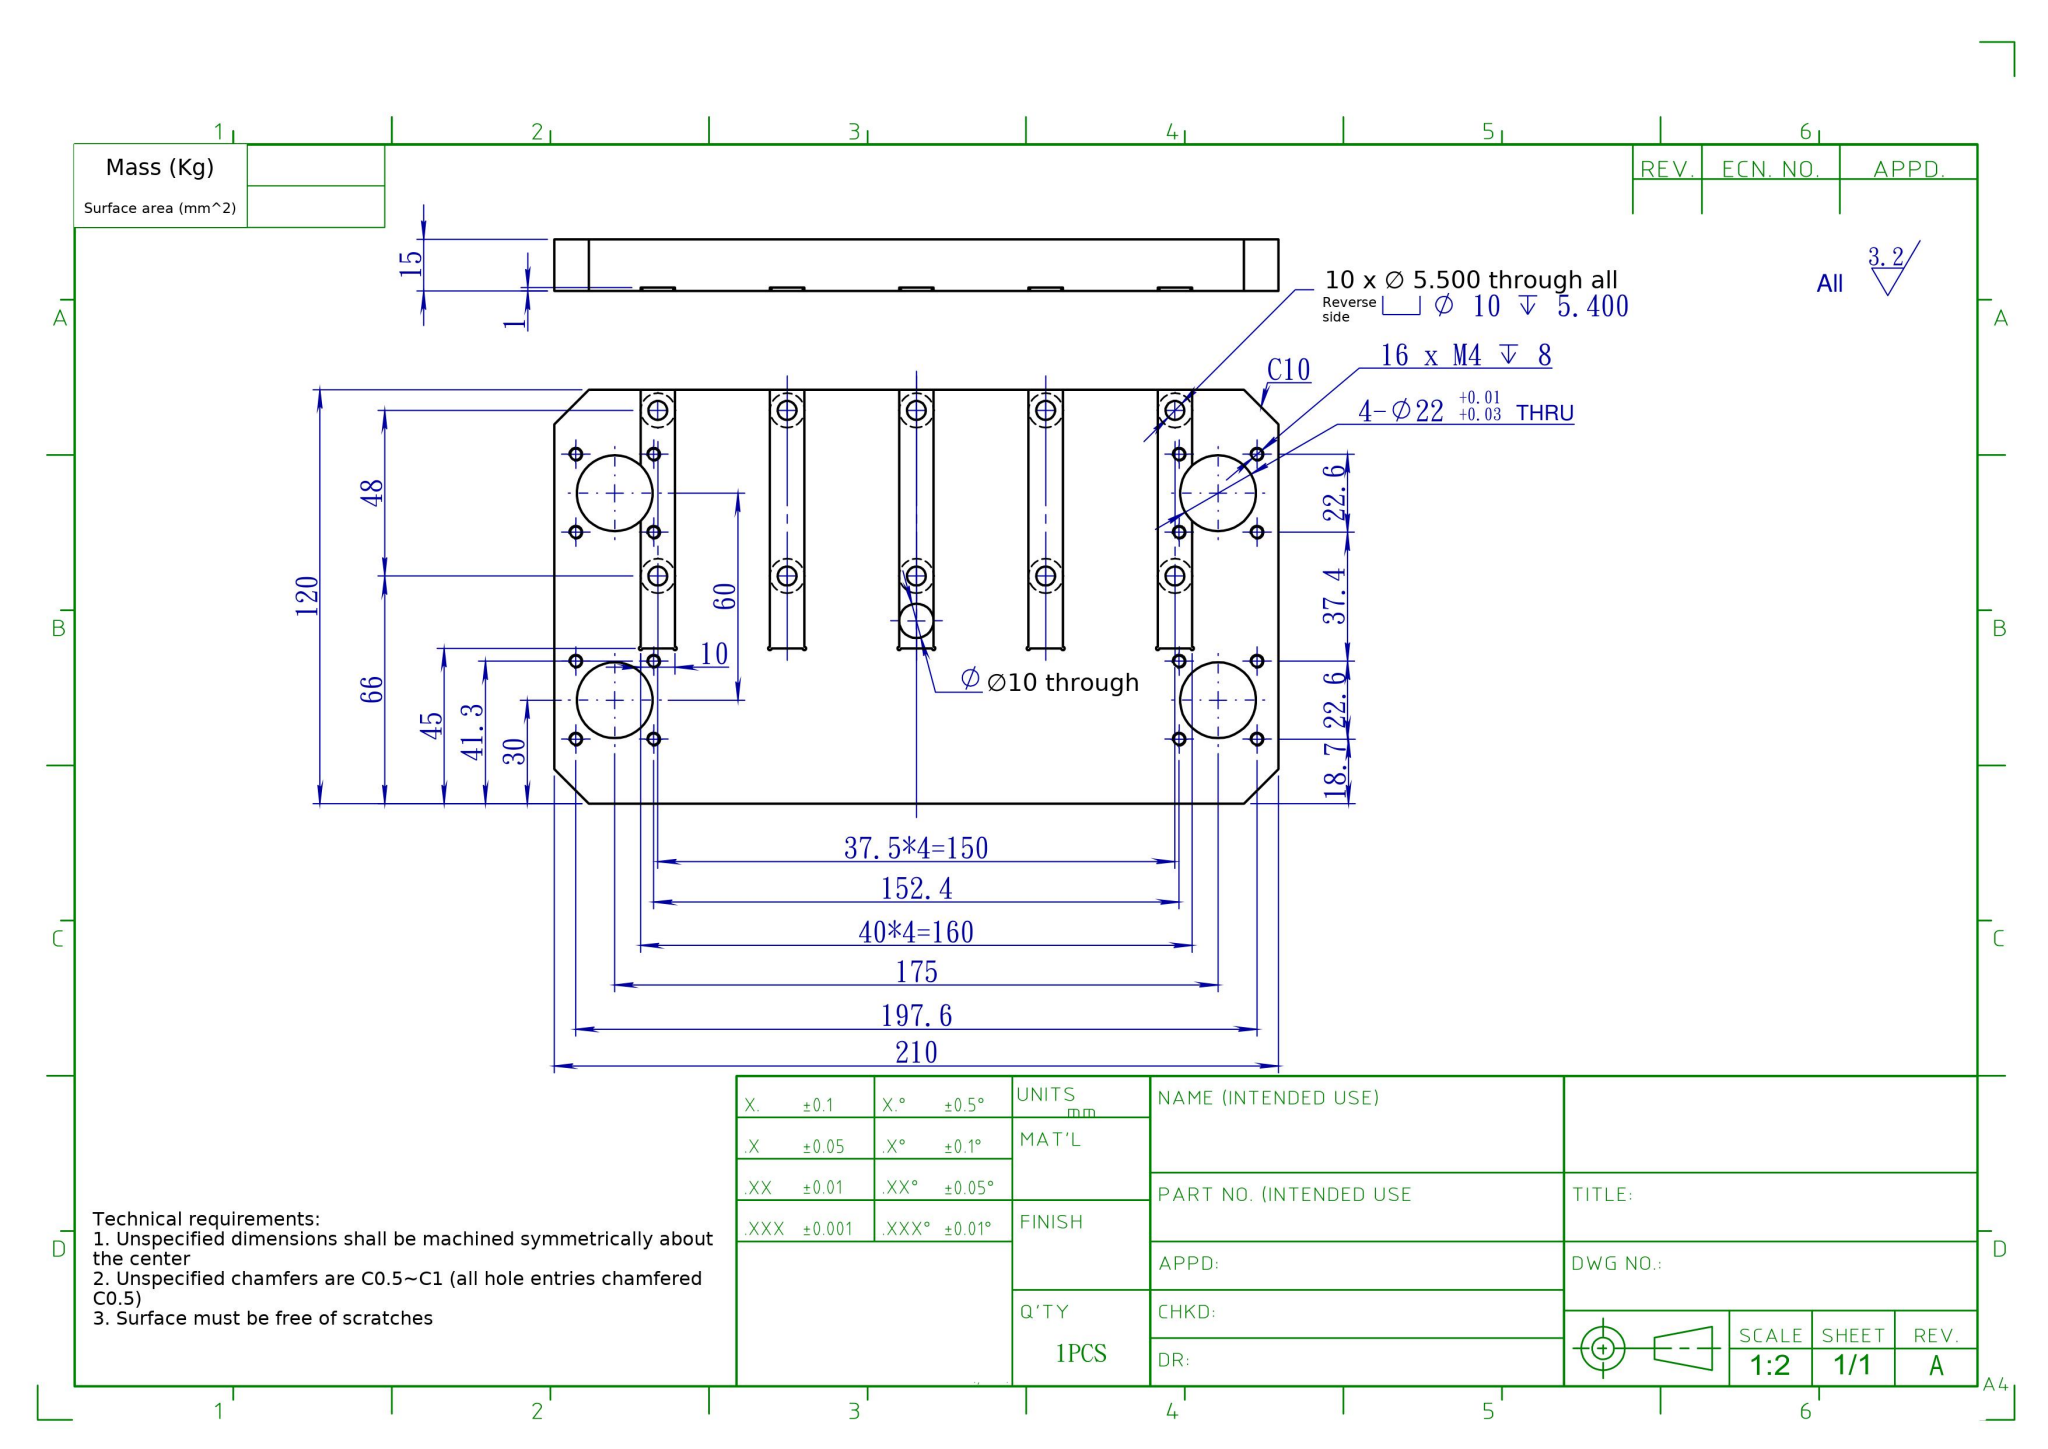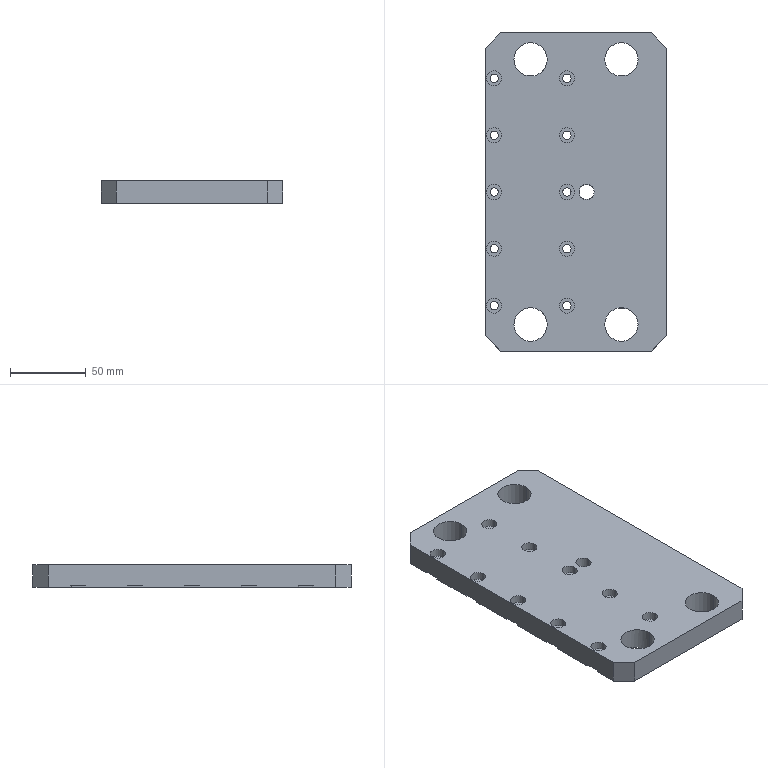Part | SolidWorks | mm | 1 solid | 167 faces | box 120 x 210 x 15 mm | volume 339737 mm3 | cylinder 92 | plane 43 | cone 32 | commonest cylinder face diameters 3.3 x32 10 x22 5.5 x20 1 x10 22 x8
build123d program:
from build123d import *

# Parameters (mm, degrees)
SKETCH1_2_W                                         = 120
SKETCH1_2_H                                         = 210
BOSS_EXTRUDE1_DEPTH                                 = 15
SKETCH2_2_R                                         = 11
CUT_EXTRUDE1_DEPTH                                  = 15
SKETCH3_2_R                                         = 5
CUT_EXTRUDE2_DEPTH                                  = 122.861
CHAMFER1_SIZE                                       = 10
CBORE_FOR_M5_HEX_SOCKET_HEAD_CAP_SCREW1_D           = 5.5
CBORE_FOR_M5_HEX_SOCKET_HEAD_CAP_SCREW1_CBORE_D     = 10
CBORE_FOR_M5_HEX_SOCKET_HEAD_CAP_SCREW1_CBORE_DEPTH = 5.4
M4_TAPPED_HOLE1_D                                   = 3.3
M4_TAPPED_HOLE1_DEPTH                               = 10.1
M4_TAPPED_HOLE1_TIP                                 = 0.9914
SKETCH6_W                                           = 75
SKETCH6_H                                           = 10
CUT_EXTRUDE6_DEPTH                                  = 1
LPATTERN1_COUNT                                     = 5
LPATTERN1_PITCH                                     = 37.5
SKETCH7_R                                           = 0.5
CUT_EXTRUDE7_DEPTH                                  = 1
LPATTERN2_COUNT                                     = 5
LPATTERN2_PITCH                                     = 37.5


with BuildPart() as part:
    # Sketch1_2 → Boss-Extrude1 (new body)
    with BuildSketch(Plane.XY):
        Rectangle(SKETCH1_2_W, SKETCH1_2_H)
    extrude(amount=BOSS_EXTRUDE1_DEPTH)

    # Sketch2_2 → Cut-Extrude1 (cut)
    with BuildSketch(Plane.XY.offset(15)):
        with Locations((-30, 87.5)):
            Circle(SKETCH2_2_R)
        with Locations((-30, -87.5)):
            Circle(SKETCH2_2_R)
        with Locations((30, -87.5)):
            Circle(SKETCH2_2_R)
        with Locations((30, 87.5)):
            Circle(SKETCH2_2_R)
    extrude(amount=-CUT_EXTRUDE1_DEPTH, mode=Mode.SUBTRACT)

    # Sketch3_2 → Cut-Extrude2 (cut, through all)
    with BuildSketch(Plane.XY.offset(15)):
        with Locations((7, 0)):
            Circle(SKETCH3_2_R)
    extrude(amount=-CUT_EXTRUDE2_DEPTH, mode=Mode.SUBTRACT)

    # Chamfer1
    chamfer1_edges = [part.edges().sort_by_distance(p)[0] for p in [
        (-60, 105, 7.5),
        (60, 105, 7.5),
        (60, -105, 7.5),
        (-60, -105, 7.5),
    ]]
    chamfer(chamfer1_edges, length=CHAMFER1_SIZE)

    # CBORE for M5 Hex Socket Head Cap Screw1 (through all)
    with Locations(Plane.XY.offset(15)):
        with Locations((-54, 75), (-6, 75), (-54, 37.5), (-6, 37.5), (-54, 0), (-6, 0), (-54, -37.5), (-6, -37.5), (-54, -75), (-6, -75)):
            CounterBoreHole(CBORE_FOR_M5_HEX_SOCKET_HEAD_CAP_SCREW1_D / 2, CBORE_FOR_M5_HEX_SOCKET_HEAD_CAP_SCREW1_CBORE_D / 2, CBORE_FOR_M5_HEX_SOCKET_HEAD_CAP_SCREW1_CBORE_DEPTH)

    # M4 Tapped Hole1
    with Locations(Plane(origin=(0, 0, 0), x_dir=(-1, 0, 0), z_dir=(0, 0, -1))):
        with Locations((-41.3, 98.8), (-41.3, 76.2), (-18.7, 98.8), (-18.7, 76.2), (18.7, 76.2), (18.7, 98.8), (41.3, 76.2), (41.3, 98.8), (41.3, -98.8), (41.3, -76.2), (18.7, -98.8), (18.7, -76.2), (-18.7, -76.2), (-18.7, -98.8), (-41.3, -76.2), (-41.3, -98.8)):
            Hole(M4_TAPPED_HOLE1_D / 2, depth=M4_TAPPED_HOLE1_DEPTH)
            with Locations((0, 0, -(M4_TAPPED_HOLE1_DEPTH + M4_TAPPED_HOLE1_TIP / 2))):  # 118° drill point
                Cone(0, M4_TAPPED_HOLE1_D / 2, M4_TAPPED_HOLE1_TIP, mode=Mode.SUBTRACT)

    # Sketch6 → Cut-Extrude6 (cut)
    with BuildSketch(Plane(origin=(0, 0, 0), x_dir=(-1, 0, 0), z_dir=(0, 0, -1))):
        with Locations((22.5, 75)):
            Rectangle(SKETCH6_W, SKETCH6_H)
    cut_extrude6 = extrude(amount=-CUT_EXTRUDE6_DEPTH, mode=Mode.SUBTRACT)

    # LPattern1: Cut-Extrude6 ×5
    with Locations(*[(0, -i * LPATTERN1_PITCH, 0) for i in range(1, LPATTERN1_COUNT)]):
        add(cut_extrude6, mode=Mode.SUBTRACT)

    # Sketch7 → Cut-Extrude7 (cut)
    with BuildSketch(Plane(origin=(0, 0, 0), x_dir=(-1, 0, 0), z_dir=(0, 0, -1))):
        with Locations((-15, 80)):
            Circle(SKETCH7_R)
        with Locations((-15, 70)):
            Circle(SKETCH7_R)
    cut_extrude7 = extrude(amount=-CUT_EXTRUDE7_DEPTH, mode=Mode.SUBTRACT)

    # LPattern2: Cut-Extrude7 ×5
    with Locations(*[(0, -i * LPATTERN2_PITCH, 0) for i in range(1, LPATTERN2_COUNT)]):
        add(cut_extrude7, mode=Mode.SUBTRACT)


solid = part.part